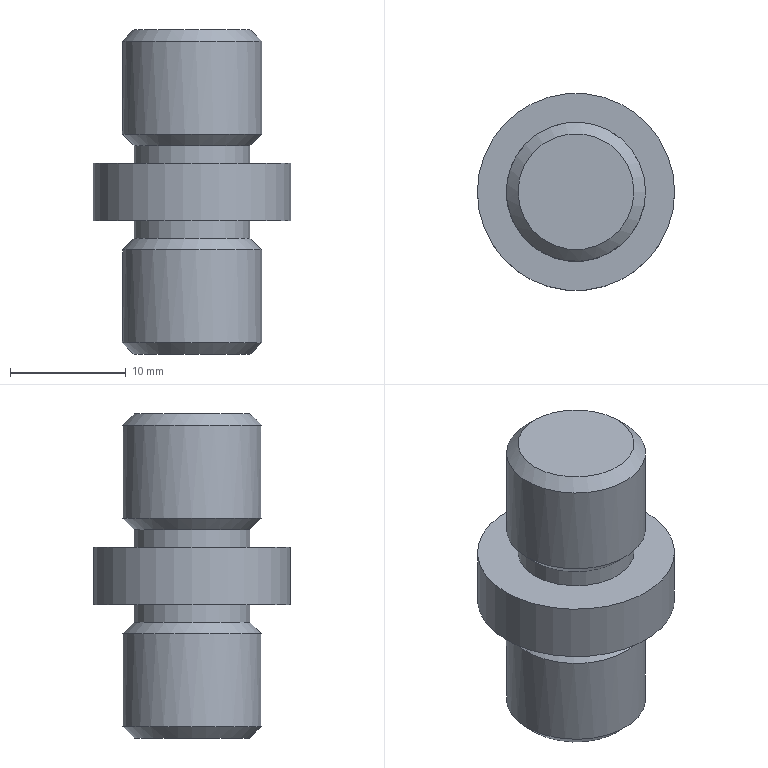Component | NX | A_LOCATING_PIN | 1 solid | 13 faces | box 17 x 17 x 28 mm | volume 3561 mm3 | cylinder 5 | plane 4 | cone 4 | commonest cylinder face diameters 12 x2 10 x2 17 x1
STEP:
#1=CARTESIAN_POINT('',(0.,0.,0.));
#2=DIRECTION('',(0.,0.,1.));
#3=DIRECTION('',(1.,0.,0.));
#4=AXIS2_PLACEMENT_3D('',#1,#2,#3);
#5=CARTESIAN_POINT('',(8.,-18.,40.5));
#6=VERTEX_POINT('',#5);
#7=CARTESIAN_POINT('',(13.,-18.,40.5));
#8=DIRECTION('',(0.,0.,-1.));
#9=DIRECTION('',(-1.,0.,0.));
#10=AXIS2_PLACEMENT_3D('',#7,#8,#9);
#11=CIRCLE('',#10,5.);
#12=CARTESIAN_POINT('',(13.,-18.,40.5));
#13=DIRECTION('',(0.,0.,-1.));
#14=DIRECTION('',(-1.,0.,0.));
#15=AXIS2_PLACEMENT_3D('',#12,#13,#14);
#16=PLANE('',#15);
#17=CARTESIAN_POINT('',(0.,0.));
#18=DIRECTION('',(1.,0.));
#19=AXIS2_PLACEMENT_2D('',#17,#18);
#20=CIRCLE('',#19,5.);
#21=(GEOMETRIC_REPRESENTATION_CONTEXT(2)PARAMETRIC_REPRESENTATION_CONTEXT()REPRESENTATION_CONTEXT('',''));
#22=DEFINITIONAL_REPRESENTATION('',(#20),#21);
#23=PCURVE('',#16,#22);
#24=CARTESIAN_POINT('',(13.,-18.,41.5));
#25=DIRECTION('',(0.,0.,1.));
#26=DIRECTION('',(1.,0.,0.));
#27=AXIS2_PLACEMENT_3D('',#24,#25,#26);
#28=CONICAL_SURFACE('',#27,6.,0.7854);
#29=CARTESIAN_POINT('',(9.425,-1.));
#30=DIRECTION('',(-1.,0.));
#31=VECTOR('',#30,1.);
#32=LINE('',#29,#31);
#33=(GEOMETRIC_REPRESENTATION_CONTEXT(2)PARAMETRIC_REPRESENTATION_CONTEXT()REPRESENTATION_CONTEXT('',''));
#34=DEFINITIONAL_REPRESENTATION('',(#32),#33);
#35=PCURVE('',#28,#34);
#36=SURFACE_CURVE('',#11,(#23,#35),.PCURVE_S1.);
#37=EDGE_CURVE('',#6,#6,#36,.T.);
#38=ORIENTED_EDGE('',*,*,#37,.T.);
#39=EDGE_LOOP('',(#38));
#40=FACE_BOUND('',#39,.T.);
#41=ADVANCED_FACE('',(#40),#16,.T.);
#42=CARTESIAN_POINT('',(7.,-18.,41.5));
#43=VERTEX_POINT('',#42);
#44=CARTESIAN_POINT('',(19.,-18.,41.5));
#45=VERTEX_POINT('',#44);
#46=CARTESIAN_POINT('',(13.,-18.,41.5));
#47=DIRECTION('',(0.,0.,1.));
#48=DIRECTION('',(-1.,0.,0.));
#49=AXIS2_PLACEMENT_3D('',#46,#47,#48);
#50=CIRCLE('',#49,6.);
#51=CARTESIAN_POINT('',(13.,-18.,40.5));
#52=DIRECTION('',(0.,0.,1.));
#53=DIRECTION('',(1.,0.,0.));
#54=AXIS2_PLACEMENT_3D('',#51,#52,#53);
#55=CYLINDRICAL_SURFACE('',#54,6.);
#56=CARTESIAN_POINT('',(3.142,1.));
#57=DIRECTION('',(1.,0.));
#58=VECTOR('',#57,1.);
#59=LINE('',#56,#58);
#60=(GEOMETRIC_REPRESENTATION_CONTEXT(2)PARAMETRIC_REPRESENTATION_CONTEXT()REPRESENTATION_CONTEXT('',''));
#61=DEFINITIONAL_REPRESENTATION('',(#59),#60);
#62=PCURVE('',#55,#61);
#63=CARTESIAN_POINT('',(3.142,0.));
#64=DIRECTION('',(1.,0.));
#65=VECTOR('',#64,1.);
#66=LINE('',#63,#65);
#67=(GEOMETRIC_REPRESENTATION_CONTEXT(2)PARAMETRIC_REPRESENTATION_CONTEXT()REPRESENTATION_CONTEXT('',''));
#68=DEFINITIONAL_REPRESENTATION('',(#66),#67);
#69=PCURVE('',#28,#68);
#70=SURFACE_CURVE('',#50,(#62,#69),.PCURVE_S1.);
#71=EDGE_CURVE('',#43,#45,#70,.T.);
#72=ORIENTED_EDGE('',*,*,#71,.T.);
#73=CARTESIAN_POINT('',(19.,-18.,49.5));
#74=VERTEX_POINT('',#73);
#75=CARTESIAN_POINT('',(19.,-18.,41.5));
#76=CARTESIAN_POINT('',(19.,-18.,49.5));
#77=B_SPLINE_CURVE_WITH_KNOTS('',1,(#75,#76),.UNSPECIFIED.,.F.,.F.,(2,2),(1.,9.),.PIECEWISE_BEZIER_KNOTS.);
#78=CARTESIAN_POINT('',(6.283,0.));
#79=DIRECTION('',(0.,1.));
#80=VECTOR('',#79,1.);
#81=LINE('',#78,#80);
#82=(GEOMETRIC_REPRESENTATION_CONTEXT(2)PARAMETRIC_REPRESENTATION_CONTEXT()REPRESENTATION_CONTEXT('',''));
#83=DEFINITIONAL_REPRESENTATION('',(#81),#82);
#84=PCURVE('',#55,#83);
#85=CARTESIAN_POINT('',(0.,0.));
#86=DIRECTION('',(0.,1.));
#87=VECTOR('',#86,1.);
#88=LINE('',#85,#87);
#89=(GEOMETRIC_REPRESENTATION_CONTEXT(2)PARAMETRIC_REPRESENTATION_CONTEXT()REPRESENTATION_CONTEXT('',''));
#90=DEFINITIONAL_REPRESENTATION('',(#88),#89);
#91=PCURVE('',#55,#90);
#92=SEAM_CURVE('',#77,(#84,#91),.PCURVE_S1.);
#93=EDGE_CURVE('',#45,#74,#92,.T.);
#94=ORIENTED_EDGE('',*,*,#93,.T.);
#95=CARTESIAN_POINT('',(13.,-18.,49.5));
#96=DIRECTION('',(0.,0.,-1.));
#97=DIRECTION('',(1.,0.,0.));
#98=AXIS2_PLACEMENT_3D('',#95,#96,#97);
#99=CIRCLE('',#98,6.);
#100=CARTESIAN_POINT('',(6.283,9.));
#101=DIRECTION('',(-1.,0.));
#102=VECTOR('',#101,1.);
#103=LINE('',#100,#102);
#104=(GEOMETRIC_REPRESENTATION_CONTEXT(2)PARAMETRIC_REPRESENTATION_CONTEXT()REPRESENTATION_CONTEXT('',''));
#105=DEFINITIONAL_REPRESENTATION('',(#103),#104);
#106=PCURVE('',#55,#105);
#107=CARTESIAN_POINT('',(13.,-18.,49.5));
#108=DIRECTION('',(0.,0.,-1.));
#109=DIRECTION('',(-1.,0.,0.));
#110=AXIS2_PLACEMENT_3D('',#107,#108,#109);
#111=CONICAL_SURFACE('',#110,6.,0.7854);
#112=CARTESIAN_POINT('',(3.142,0.));
#113=DIRECTION('',(1.,0.));
#114=VECTOR('',#113,1.);
#115=LINE('',#112,#114);
#116=(GEOMETRIC_REPRESENTATION_CONTEXT(2)PARAMETRIC_REPRESENTATION_CONTEXT()REPRESENTATION_CONTEXT('',''));
#117=DEFINITIONAL_REPRESENTATION('',(#115),#116);
#118=PCURVE('',#111,#117);
#119=SURFACE_CURVE('',#99,(#106,#118),.PCURVE_S1.);
#120=EDGE_CURVE('',#74,#74,#119,.T.);
#121=ORIENTED_EDGE('',*,*,#120,.T.);
#122=ORIENTED_EDGE('',*,*,#93,.F.);
#123=CARTESIAN_POINT('',(13.,-18.,41.5));
#124=DIRECTION('',(0.,0.,1.));
#125=DIRECTION('',(-1.,0.,0.));
#126=AXIS2_PLACEMENT_3D('',#123,#124,#125);
#127=CIRCLE('',#126,6.);
#128=CARTESIAN_POINT('',(-3.142,1.));
#129=DIRECTION('',(1.,0.));
#130=VECTOR('',#129,1.);
#131=LINE('',#128,#130);
#132=(GEOMETRIC_REPRESENTATION_CONTEXT(2)PARAMETRIC_REPRESENTATION_CONTEXT()REPRESENTATION_CONTEXT('',''));
#133=DEFINITIONAL_REPRESENTATION('',(#131),#132);
#134=PCURVE('',#55,#133);
#135=CARTESIAN_POINT('',(3.142,0.));
#136=DIRECTION('',(1.,0.));
#137=VECTOR('',#136,1.);
#138=LINE('',#135,#137);
#139=(GEOMETRIC_REPRESENTATION_CONTEXT(2)PARAMETRIC_REPRESENTATION_CONTEXT()REPRESENTATION_CONTEXT('',''));
#140=DEFINITIONAL_REPRESENTATION('',(#138),#139);
#141=PCURVE('',#28,#140);
#142=SURFACE_CURVE('',#127,(#134,#141),.PCURVE_S1.);
#143=EDGE_CURVE('',#45,#43,#142,.T.);
#144=ORIENTED_EDGE('',*,*,#143,.T.);
#145=EDGE_LOOP('',(#72,#94,#121,#122,#144));
#146=FACE_BOUND('',#145,.T.);
#147=ADVANCED_FACE('',(#146),#55,.T.);
#148=CARTESIAN_POINT('',(18.,-18.,52.));
#149=VERTEX_POINT('',#148);
#150=CARTESIAN_POINT('',(8.,-18.,52.));
#151=VERTEX_POINT('',#150);
#152=CARTESIAN_POINT('',(13.,-18.,52.));
#153=DIRECTION('',(0.,0.,1.));
#154=DIRECTION('',(-1.,0.,0.));
#155=AXIS2_PLACEMENT_3D('',#152,#153,#154);
#156=CIRCLE('',#155,5.);
#157=CARTESIAN_POINT('',(13.,-18.,50.5));
#158=DIRECTION('',(0.,0.,1.));
#159=DIRECTION('',(1.,0.,0.));
#160=AXIS2_PLACEMENT_3D('',#157,#158,#159);
#161=CYLINDRICAL_SURFACE('',#160,5.);
#162=CARTESIAN_POINT('',(-3.142,1.5));
#163=DIRECTION('',(1.,0.));
#164=VECTOR('',#163,1.);
#165=LINE('',#162,#164);
#166=(GEOMETRIC_REPRESENTATION_CONTEXT(2)PARAMETRIC_REPRESENTATION_CONTEXT()REPRESENTATION_CONTEXT('',''));
#167=DEFINITIONAL_REPRESENTATION('',(#165),#166);
#168=PCURVE('',#161,#167);
#169=CARTESIAN_POINT('',(13.,-18.,52.));
#170=DIRECTION('',(0.,0.,-1.));
#171=DIRECTION('',(-1.,0.,0.));
#172=AXIS2_PLACEMENT_3D('',#169,#170,#171);
#173=PLANE('',#172);
#174=CARTESIAN_POINT('',(5.,0.));
#175=CARTESIAN_POINT('',(5.,-8.66));
#176=CARTESIAN_POINT('',(-2.5,-4.33));
#177=CARTESIAN_POINT('',(-10.,-0.));
#178=CARTESIAN_POINT('',(-2.5,4.33));
#179=CARTESIAN_POINT('',(5.,8.66));
#180=CARTESIAN_POINT('',(5.,0.));
#181=(BOUNDED_CURVE()B_SPLINE_CURVE(2,(#174,#175,#176,#177,#178,#179,#180),.UNSPECIFIED.,.T.,.F.)B_SPLINE_CURVE_WITH_KNOTS((1,2,2,2,2,1),(-2.094,0.,2.094,4.189,6.283,8.378),.UNSPECIFIED.)CURVE()GEOMETRIC_REPRESENTATION_ITEM()RATIONAL_B_SPLINE_CURVE((1.,0.5,1.,0.5,1.,0.5,1.))REPRESENTATION_ITEM(''));
#182=(GEOMETRIC_REPRESENTATION_CONTEXT(2)PARAMETRIC_REPRESENTATION_CONTEXT()REPRESENTATION_CONTEXT('',''));
#183=DEFINITIONAL_REPRESENTATION('',(#181),#182);
#184=PCURVE('',#173,#183);
#185=SURFACE_CURVE('',#156,(#168,#184),.PCURVE_S1.);
#186=EDGE_CURVE('',#149,#151,#185,.T.);
#187=ORIENTED_EDGE('',*,*,#186,.F.);
#188=CARTESIAN_POINT('',(18.,-18.,50.5));
#189=VERTEX_POINT('',#188);
#190=CARTESIAN_POINT('',(18.,-18.,50.5));
#191=CARTESIAN_POINT('',(18.,-18.,52.));
#192=B_SPLINE_CURVE_WITH_KNOTS('',1,(#190,#191),.UNSPECIFIED.,.F.,.F.,(2,2),(0.,1.5),.PIECEWISE_BEZIER_KNOTS.);
#193=CARTESIAN_POINT('',(0.,0.));
#194=DIRECTION('',(0.,1.));
#195=VECTOR('',#194,1.);
#196=LINE('',#193,#195);
#197=(GEOMETRIC_REPRESENTATION_CONTEXT(2)PARAMETRIC_REPRESENTATION_CONTEXT()REPRESENTATION_CONTEXT('',''));
#198=DEFINITIONAL_REPRESENTATION('',(#196),#197);
#199=PCURVE('',#161,#198);
#200=CARTESIAN_POINT('',(6.283,0.));
#201=DIRECTION('',(0.,1.));
#202=VECTOR('',#201,1.);
#203=LINE('',#200,#202);
#204=(GEOMETRIC_REPRESENTATION_CONTEXT(2)PARAMETRIC_REPRESENTATION_CONTEXT()REPRESENTATION_CONTEXT('',''));
#205=DEFINITIONAL_REPRESENTATION('',(#203),#204);
#206=PCURVE('',#161,#205);
#207=SEAM_CURVE('',#192,(#199,#206),.PCURVE_S1.);
#208=EDGE_CURVE('',#189,#149,#207,.T.);
#209=ORIENTED_EDGE('',*,*,#208,.F.);
#210=CARTESIAN_POINT('',(13.,-18.,50.5));
#211=DIRECTION('',(0.,0.,1.));
#212=DIRECTION('',(1.,0.,0.));
#213=AXIS2_PLACEMENT_3D('',#210,#211,#212);
#214=CIRCLE('',#213,5.);
#215=CARTESIAN_POINT('',(0.,0.));
#216=DIRECTION('',(1.,0.));
#217=VECTOR('',#216,1.);
#218=LINE('',#215,#217);
#219=(GEOMETRIC_REPRESENTATION_CONTEXT(2)PARAMETRIC_REPRESENTATION_CONTEXT()REPRESENTATION_CONTEXT('',''));
#220=DEFINITIONAL_REPRESENTATION('',(#218),#219);
#221=PCURVE('',#161,#220);
#222=CARTESIAN_POINT('',(9.425,-1.));
#223=DIRECTION('',(-1.,0.));
#224=VECTOR('',#223,1.);
#225=LINE('',#222,#224);
#226=(GEOMETRIC_REPRESENTATION_CONTEXT(2)PARAMETRIC_REPRESENTATION_CONTEXT()REPRESENTATION_CONTEXT('',''));
#227=DEFINITIONAL_REPRESENTATION('',(#225),#226);
#228=PCURVE('',#111,#227);
#229=SURFACE_CURVE('',#214,(#221,#228),.PCURVE_S1.);
#230=EDGE_CURVE('',#189,#189,#229,.T.);
#231=ORIENTED_EDGE('',*,*,#230,.T.);
#232=ORIENTED_EDGE('',*,*,#208,.T.);
#233=CARTESIAN_POINT('',(13.,-18.,52.));
#234=DIRECTION('',(0.,0.,1.));
#235=DIRECTION('',(-1.,0.,0.));
#236=AXIS2_PLACEMENT_3D('',#233,#234,#235);
#237=CIRCLE('',#236,5.);
#238=CARTESIAN_POINT('',(3.142,1.5));
#239=DIRECTION('',(1.,0.));
#240=VECTOR('',#239,1.);
#241=LINE('',#238,#240);
#242=(GEOMETRIC_REPRESENTATION_CONTEXT(2)PARAMETRIC_REPRESENTATION_CONTEXT()REPRESENTATION_CONTEXT('',''));
#243=DEFINITIONAL_REPRESENTATION('',(#241),#242);
#244=PCURVE('',#161,#243);
#245=CARTESIAN_POINT('',(5.,0.));
#246=CARTESIAN_POINT('',(5.,-8.66));
#247=CARTESIAN_POINT('',(-2.5,-4.33));
#248=CARTESIAN_POINT('',(-10.,-0.));
#249=CARTESIAN_POINT('',(-2.5,4.33));
#250=CARTESIAN_POINT('',(5.,8.66));
#251=CARTESIAN_POINT('',(5.,0.));
#252=(BOUNDED_CURVE()B_SPLINE_CURVE(2,(#245,#246,#247,#248,#249,#250,#251),.UNSPECIFIED.,.T.,.F.)B_SPLINE_CURVE_WITH_KNOTS((1,2,2,2,2,1),(-2.094,0.,2.094,4.189,6.283,8.378),.UNSPECIFIED.)CURVE()GEOMETRIC_REPRESENTATION_ITEM()RATIONAL_B_SPLINE_CURVE((1.,0.5,1.,0.5,1.,0.5,1.))REPRESENTATION_ITEM(''));
#253=(GEOMETRIC_REPRESENTATION_CONTEXT(2)PARAMETRIC_REPRESENTATION_CONTEXT()REPRESENTATION_CONTEXT('',''));
#254=DEFINITIONAL_REPRESENTATION('',(#252),#253);
#255=PCURVE('',#173,#254);
#256=SURFACE_CURVE('',#237,(#244,#255),.PCURVE_S1.);
#257=EDGE_CURVE('',#151,#149,#256,.T.);
#258=ORIENTED_EDGE('',*,*,#257,.F.);
#259=EDGE_LOOP('',(#187,#209,#231,#232,#258));
#260=FACE_BOUND('',#259,.T.);
#261=ADVANCED_FACE('',(#260),#161,.T.);
#262=CARTESIAN_POINT('',(18.,-18.,57.));
#263=VERTEX_POINT('',#262);
#264=CARTESIAN_POINT('',(13.,-18.,57.));
#265=DIRECTION('',(0.,0.,1.));
#266=DIRECTION('',(1.,0.,0.));
#267=AXIS2_PLACEMENT_3D('',#264,#265,#266);
#268=CIRCLE('',#267,5.);
#269=CARTESIAN_POINT('',(13.,-18.,57.));
#270=DIRECTION('',(0.,0.,1.));
#271=DIRECTION('',(1.,0.,0.));
#272=AXIS2_PLACEMENT_3D('',#269,#270,#271);
#273=PLANE('',#272);
#274=CARTESIAN_POINT('',(0.,0.));
#275=DIRECTION('',(1.,0.));
#276=AXIS2_PLACEMENT_2D('',#274,#275);
#277=CIRCLE('',#276,5.);
#278=(GEOMETRIC_REPRESENTATION_CONTEXT(2)PARAMETRIC_REPRESENTATION_CONTEXT()REPRESENTATION_CONTEXT('',''));
#279=DEFINITIONAL_REPRESENTATION('',(#277),#278);
#280=PCURVE('',#273,#279);
#281=CARTESIAN_POINT('',(13.,-18.,57.));
#282=DIRECTION('',(0.,0.,1.));
#283=DIRECTION('',(1.,0.,0.));
#284=AXIS2_PLACEMENT_3D('',#281,#282,#283);
#285=CYLINDRICAL_SURFACE('',#284,5.);
#286=CARTESIAN_POINT('',(0.,0.));
#287=DIRECTION('',(1.,0.));
#288=VECTOR('',#287,1.);
#289=LINE('',#286,#288);
#290=(GEOMETRIC_REPRESENTATION_CONTEXT(2)PARAMETRIC_REPRESENTATION_CONTEXT()REPRESENTATION_CONTEXT('',''));
#291=DEFINITIONAL_REPRESENTATION('',(#289),#290);
#292=PCURVE('',#285,#291);
#293=SURFACE_CURVE('',#268,(#280,#292),.PCURVE_S1.);
#294=EDGE_CURVE('',#263,#263,#293,.T.);
#295=ORIENTED_EDGE('',*,*,#294,.F.);
#296=EDGE_LOOP('',(#295));
#297=FACE_BOUND('',#296,.T.);
#298=CARTESIAN_POINT('',(21.5,-18.,57.));
#299=VERTEX_POINT('',#298);
#300=CARTESIAN_POINT('',(13.,-18.,57.));
#301=DIRECTION('',(0.,0.,-1.));
#302=DIRECTION('',(1.,0.,0.));
#303=AXIS2_PLACEMENT_3D('',#300,#301,#302);
#304=CIRCLE('',#303,8.5);
#305=CARTESIAN_POINT('',(8.5,0.));
#306=CARTESIAN_POINT('',(8.5,-14.722));
#307=CARTESIAN_POINT('',(-4.25,-7.361));
#308=CARTESIAN_POINT('',(-17.,-0.));
#309=CARTESIAN_POINT('',(-4.25,7.361));
#310=CARTESIAN_POINT('',(8.5,14.722));
#311=CARTESIAN_POINT('',(8.5,0.));
#312=(BOUNDED_CURVE()B_SPLINE_CURVE(2,(#305,#306,#307,#308,#309,#310,#311),.UNSPECIFIED.,.T.,.F.)B_SPLINE_CURVE_WITH_KNOTS((1,2,2,2,2,1),(-2.094,0.,2.094,4.189,6.283,8.378),.UNSPECIFIED.)CURVE()GEOMETRIC_REPRESENTATION_ITEM()RATIONAL_B_SPLINE_CURVE((1.,0.5,1.,0.5,1.,0.5,1.))REPRESENTATION_ITEM(''));
#313=(GEOMETRIC_REPRESENTATION_CONTEXT(2)PARAMETRIC_REPRESENTATION_CONTEXT()REPRESENTATION_CONTEXT('',''));
#314=DEFINITIONAL_REPRESENTATION('',(#312),#313);
#315=PCURVE('',#273,#314);
#316=CARTESIAN_POINT('',(13.,-18.,52.));
#317=DIRECTION('',(0.,0.,1.));
#318=DIRECTION('',(1.,0.,0.));
#319=AXIS2_PLACEMENT_3D('',#316,#317,#318);
#320=CYLINDRICAL_SURFACE('',#319,8.5);
#321=CARTESIAN_POINT('',(6.283,5.));
#322=DIRECTION('',(-1.,0.));
#323=VECTOR('',#322,1.);
#324=LINE('',#321,#323);
#325=(GEOMETRIC_REPRESENTATION_CONTEXT(2)PARAMETRIC_REPRESENTATION_CONTEXT()REPRESENTATION_CONTEXT('',''));
#326=DEFINITIONAL_REPRESENTATION('',(#324),#325);
#327=PCURVE('',#320,#326);
#328=SURFACE_CURVE('',#304,(#315,#327),.PCURVE_S1.);
#329=EDGE_CURVE('',#299,#299,#328,.T.);
#330=ORIENTED_EDGE('',*,*,#329,.F.);
#331=EDGE_LOOP('',(#330));
#332=FACE_BOUND('',#331,.T.);
#333=ADVANCED_FACE('',(#297,#332),#273,.T.);
#334=ORIENTED_EDGE('',*,*,#257,.T.);
#335=ORIENTED_EDGE('',*,*,#186,.T.);
#336=EDGE_LOOP('',(#334,#335));
#337=FACE_BOUND('',#336,.T.);
#338=CARTESIAN_POINT('',(21.5,-18.,52.));
#339=VERTEX_POINT('',#338);
#340=CARTESIAN_POINT('',(13.,-18.,52.));
#341=DIRECTION('',(0.,0.,1.));
#342=DIRECTION('',(1.,0.,0.));
#343=AXIS2_PLACEMENT_3D('',#340,#341,#342);
#344=CIRCLE('',#343,8.5);
#345=CARTESIAN_POINT('',(-8.5,0.));
#346=CARTESIAN_POINT('',(-8.5,14.722));
#347=CARTESIAN_POINT('',(4.25,7.361));
#348=CARTESIAN_POINT('',(17.,0.));
#349=CARTESIAN_POINT('',(4.25,-7.361));
#350=CARTESIAN_POINT('',(-8.5,-14.722));
#351=CARTESIAN_POINT('',(-8.5,0.));
#352=(BOUNDED_CURVE()B_SPLINE_CURVE(2,(#345,#346,#347,#348,#349,#350,#351),.UNSPECIFIED.,.T.,.F.)B_SPLINE_CURVE_WITH_KNOTS((1,2,2,2,2,1),(-2.094,0.,2.094,4.189,6.283,8.378),.UNSPECIFIED.)CURVE()GEOMETRIC_REPRESENTATION_ITEM()RATIONAL_B_SPLINE_CURVE((1.,0.5,1.,0.5,1.,0.5,1.))REPRESENTATION_ITEM(''));
#353=(GEOMETRIC_REPRESENTATION_CONTEXT(2)PARAMETRIC_REPRESENTATION_CONTEXT()REPRESENTATION_CONTEXT('',''));
#354=DEFINITIONAL_REPRESENTATION('',(#352),#353);
#355=PCURVE('',#173,#354);
#356=CARTESIAN_POINT('',(0.,0.));
#357=DIRECTION('',(1.,0.));
#358=VECTOR('',#357,1.);
#359=LINE('',#356,#358);
#360=(GEOMETRIC_REPRESENTATION_CONTEXT(2)PARAMETRIC_REPRESENTATION_CONTEXT()REPRESENTATION_CONTEXT('',''));
#361=DEFINITIONAL_REPRESENTATION('',(#359),#360);
#362=PCURVE('',#320,#361);
#363=SURFACE_CURVE('',#344,(#355,#362),.PCURVE_S1.);
#364=EDGE_CURVE('',#339,#339,#363,.T.);
#365=ORIENTED_EDGE('',*,*,#364,.F.);
#366=EDGE_LOOP('',(#365));
#367=FACE_BOUND('',#366,.T.);
#368=ADVANCED_FACE('',(#337,#367),#173,.T.);
#369=ORIENTED_EDGE('',*,*,#329,.T.);
#370=CARTESIAN_POINT('',(21.5,-18.,52.));
#371=CARTESIAN_POINT('',(21.5,-18.,57.));
#372=B_SPLINE_CURVE_WITH_KNOTS('',1,(#370,#371),.UNSPECIFIED.,.F.,.F.,(2,2),(0.,5.),.PIECEWISE_BEZIER_KNOTS.);
#373=CARTESIAN_POINT('',(0.,0.));
#374=DIRECTION('',(0.,1.));
#375=VECTOR('',#374,1.);
#376=LINE('',#373,#375);
#377=(GEOMETRIC_REPRESENTATION_CONTEXT(2)PARAMETRIC_REPRESENTATION_CONTEXT()REPRESENTATION_CONTEXT('',''));
#378=DEFINITIONAL_REPRESENTATION('',(#376),#377);
#379=PCURVE('',#320,#378);
#380=CARTESIAN_POINT('',(6.283,0.));
#381=DIRECTION('',(0.,1.));
#382=VECTOR('',#381,1.);
#383=LINE('',#380,#382);
#384=(GEOMETRIC_REPRESENTATION_CONTEXT(2)PARAMETRIC_REPRESENTATION_CONTEXT()REPRESENTATION_CONTEXT('',''));
#385=DEFINITIONAL_REPRESENTATION('',(#383),#384);
#386=PCURVE('',#320,#385);
#387=SEAM_CURVE('',#372,(#379,#386),.PCURVE_S1.);
#388=EDGE_CURVE('',#339,#299,#387,.T.);
#389=ORIENTED_EDGE('',*,*,#388,.F.);
#390=ORIENTED_EDGE('',*,*,#364,.T.);
#391=ORIENTED_EDGE('',*,*,#388,.T.);
#392=EDGE_LOOP('',(#369,#389,#390,#391));
#393=FACE_BOUND('',#392,.T.);
#394=ADVANCED_FACE('',(#393),#320,.T.);
#395=CARTESIAN_POINT('',(18.,-18.,58.5));
#396=VERTEX_POINT('',#395);
#397=CARTESIAN_POINT('',(8.,-18.,58.5));
#398=VERTEX_POINT('',#397);
#399=CARTESIAN_POINT('',(13.,-18.,58.5));
#400=DIRECTION('',(0.,0.,1.));
#401=DIRECTION('',(-1.,0.,0.));
#402=AXIS2_PLACEMENT_3D('',#399,#400,#401);
#403=CIRCLE('',#402,5.);
#404=CARTESIAN_POINT('',(-3.142,1.5));
#405=DIRECTION('',(1.,0.));
#406=VECTOR('',#405,1.);
#407=LINE('',#404,#406);
#408=(GEOMETRIC_REPRESENTATION_CONTEXT(2)PARAMETRIC_REPRESENTATION_CONTEXT()REPRESENTATION_CONTEXT('',''));
#409=DEFINITIONAL_REPRESENTATION('',(#407),#408);
#410=PCURVE('',#285,#409);
#411=CARTESIAN_POINT('',(13.,-18.,59.5));
#412=DIRECTION('',(0.,0.,1.));
#413=DIRECTION('',(1.,0.,0.));
#414=AXIS2_PLACEMENT_3D('',#411,#412,#413);
#415=CONICAL_SURFACE('',#414,6.,0.7854);
#416=CARTESIAN_POINT('',(-3.142,-1.));
#417=DIRECTION('',(1.,0.));
#418=VECTOR('',#417,1.);
#419=LINE('',#416,#418);
#420=(GEOMETRIC_REPRESENTATION_CONTEXT(2)PARAMETRIC_REPRESENTATION_CONTEXT()REPRESENTATION_CONTEXT('',''));
#421=DEFINITIONAL_REPRESENTATION('',(#419),#420);
#422=PCURVE('',#415,#421);
#423=SURFACE_CURVE('',#403,(#410,#422),.PCURVE_S1.);
#424=EDGE_CURVE('',#396,#398,#423,.T.);
#425=ORIENTED_EDGE('',*,*,#424,.F.);
#426=CARTESIAN_POINT('',(18.,-18.,57.));
#427=CARTESIAN_POINT('',(18.,-18.,58.5));
#428=B_SPLINE_CURVE_WITH_KNOTS('',1,(#426,#427),.UNSPECIFIED.,.F.,.F.,(2,2),(0.,1.5),.PIECEWISE_BEZIER_KNOTS.);
#429=CARTESIAN_POINT('',(0.,0.));
#430=DIRECTION('',(0.,1.));
#431=VECTOR('',#430,1.);
#432=LINE('',#429,#431);
#433=(GEOMETRIC_REPRESENTATION_CONTEXT(2)PARAMETRIC_REPRESENTATION_CONTEXT()REPRESENTATION_CONTEXT('',''));
#434=DEFINITIONAL_REPRESENTATION('',(#432),#433);
#435=PCURVE('',#285,#434);
#436=CARTESIAN_POINT('',(6.283,0.));
#437=DIRECTION('',(0.,1.));
#438=VECTOR('',#437,1.);
#439=LINE('',#436,#438);
#440=(GEOMETRIC_REPRESENTATION_CONTEXT(2)PARAMETRIC_REPRESENTATION_CONTEXT()REPRESENTATION_CONTEXT('',''));
#441=DEFINITIONAL_REPRESENTATION('',(#439),#440);
#442=PCURVE('',#285,#441);
#443=SEAM_CURVE('',#428,(#435,#442),.PCURVE_S1.);
#444=EDGE_CURVE('',#263,#396,#443,.T.);
#445=ORIENTED_EDGE('',*,*,#444,.F.);
#446=ORIENTED_EDGE('',*,*,#294,.T.);
#447=ORIENTED_EDGE('',*,*,#444,.T.);
#448=CARTESIAN_POINT('',(13.,-18.,58.5));
#449=DIRECTION('',(0.,0.,1.));
#450=DIRECTION('',(-1.,0.,0.));
#451=AXIS2_PLACEMENT_3D('',#448,#449,#450);
#452=CIRCLE('',#451,5.);
#453=CARTESIAN_POINT('',(3.142,1.5));
#454=DIRECTION('',(1.,0.));
#455=VECTOR('',#454,1.);
#456=LINE('',#453,#455);
#457=(GEOMETRIC_REPRESENTATION_CONTEXT(2)PARAMETRIC_REPRESENTATION_CONTEXT()REPRESENTATION_CONTEXT('',''));
#458=DEFINITIONAL_REPRESENTATION('',(#456),#457);
#459=PCURVE('',#285,#458);
#460=CARTESIAN_POINT('',(3.142,-1.));
#461=DIRECTION('',(1.,0.));
#462=VECTOR('',#461,1.);
#463=LINE('',#460,#462);
#464=(GEOMETRIC_REPRESENTATION_CONTEXT(2)PARAMETRIC_REPRESENTATION_CONTEXT()REPRESENTATION_CONTEXT('',''));
#465=DEFINITIONAL_REPRESENTATION('',(#463),#464);
#466=PCURVE('',#415,#465);
#467=SURFACE_CURVE('',#452,(#459,#466),.PCURVE_S1.);
#468=EDGE_CURVE('',#398,#396,#467,.T.);
#469=ORIENTED_EDGE('',*,*,#468,.F.);
#470=EDGE_LOOP('',(#425,#445,#446,#447,#469));
#471=FACE_BOUND('',#470,.T.);
#472=ADVANCED_FACE('',(#471),#285,.T.);
#473=CARTESIAN_POINT('',(18.,-18.,68.5));
#474=VERTEX_POINT('',#473);
#475=CARTESIAN_POINT('',(13.,-18.,68.5));
#476=DIRECTION('',(0.,0.,1.));
#477=DIRECTION('',(1.,0.,0.));
#478=AXIS2_PLACEMENT_3D('',#475,#476,#477);
#479=CIRCLE('',#478,5.);
#480=CARTESIAN_POINT('',(13.,-18.,68.5));
#481=DIRECTION('',(0.,0.,1.));
#482=DIRECTION('',(1.,0.,0.));
#483=AXIS2_PLACEMENT_3D('',#480,#481,#482);
#484=PLANE('',#483);
#485=CARTESIAN_POINT('',(0.,0.));
#486=DIRECTION('',(1.,0.));
#487=AXIS2_PLACEMENT_2D('',#485,#486);
#488=CIRCLE('',#487,5.);
#489=(GEOMETRIC_REPRESENTATION_CONTEXT(2)PARAMETRIC_REPRESENTATION_CONTEXT()REPRESENTATION_CONTEXT('',''));
#490=DEFINITIONAL_REPRESENTATION('',(#488),#489);
#491=PCURVE('',#484,#490);
#492=CARTESIAN_POINT('',(13.,-18.,67.5));
#493=DIRECTION('',(0.,0.,-1.));
#494=DIRECTION('',(-1.,0.,0.));
#495=AXIS2_PLACEMENT_3D('',#492,#493,#494);
#496=CONICAL_SURFACE('',#495,6.,0.7854);
#497=CARTESIAN_POINT('',(9.425,-1.));
#498=DIRECTION('',(-1.,0.));
#499=VECTOR('',#498,1.);
#500=LINE('',#497,#499);
#501=(GEOMETRIC_REPRESENTATION_CONTEXT(2)PARAMETRIC_REPRESENTATION_CONTEXT()REPRESENTATION_CONTEXT('',''));
#502=DEFINITIONAL_REPRESENTATION('',(#500),#501);
#503=PCURVE('',#496,#502);
#504=SURFACE_CURVE('',#479,(#491,#503),.PCURVE_S1.);
#505=EDGE_CURVE('',#474,#474,#504,.T.);
#506=ORIENTED_EDGE('',*,*,#505,.T.);
#507=EDGE_LOOP('',(#506));
#508=FACE_BOUND('',#507,.T.);
#509=ADVANCED_FACE('',(#508),#484,.T.);
#510=CARTESIAN_POINT('',(7.,-18.,59.5));
#511=VERTEX_POINT('',#510);
#512=CARTESIAN_POINT('',(19.,-18.,59.5));
#513=VERTEX_POINT('',#512);
#514=CARTESIAN_POINT('',(13.,-18.,59.5));
#515=DIRECTION('',(0.,0.,1.));
#516=DIRECTION('',(-1.,0.,0.));
#517=AXIS2_PLACEMENT_3D('',#514,#515,#516);
#518=CIRCLE('',#517,6.);
#519=CARTESIAN_POINT('',(13.,-18.,58.5));
#520=DIRECTION('',(0.,0.,1.));
#521=DIRECTION('',(1.,0.,0.));
#522=AXIS2_PLACEMENT_3D('',#519,#520,#521);
#523=CYLINDRICAL_SURFACE('',#522,6.);
#524=CARTESIAN_POINT('',(3.142,1.));
#525=DIRECTION('',(1.,0.));
#526=VECTOR('',#525,1.);
#527=LINE('',#524,#526);
#528=(GEOMETRIC_REPRESENTATION_CONTEXT(2)PARAMETRIC_REPRESENTATION_CONTEXT()REPRESENTATION_CONTEXT('',''));
#529=DEFINITIONAL_REPRESENTATION('',(#527),#528);
#530=PCURVE('',#523,#529);
#531=CARTESIAN_POINT('',(3.142,0.));
#532=DIRECTION('',(1.,0.));
#533=VECTOR('',#532,1.);
#534=LINE('',#531,#533);
#535=(GEOMETRIC_REPRESENTATION_CONTEXT(2)PARAMETRIC_REPRESENTATION_CONTEXT()REPRESENTATION_CONTEXT('',''));
#536=DEFINITIONAL_REPRESENTATION('',(#534),#535);
#537=PCURVE('',#415,#536);
#538=SURFACE_CURVE('',#518,(#530,#537),.PCURVE_S1.);
#539=EDGE_CURVE('',#511,#513,#538,.T.);
#540=ORIENTED_EDGE('',*,*,#539,.T.);
#541=CARTESIAN_POINT('',(19.,-18.,67.5));
#542=VERTEX_POINT('',#541);
#543=CARTESIAN_POINT('',(19.,-18.,59.5));
#544=CARTESIAN_POINT('',(19.,-18.,67.5));
#545=B_SPLINE_CURVE_WITH_KNOTS('',1,(#543,#544),.UNSPECIFIED.,.F.,.F.,(2,2),(1.,9.),.PIECEWISE_BEZIER_KNOTS.);
#546=CARTESIAN_POINT('',(6.283,0.));
#547=DIRECTION('',(0.,1.));
#548=VECTOR('',#547,1.);
#549=LINE('',#546,#548);
#550=(GEOMETRIC_REPRESENTATION_CONTEXT(2)PARAMETRIC_REPRESENTATION_CONTEXT()REPRESENTATION_CONTEXT('',''));
#551=DEFINITIONAL_REPRESENTATION('',(#549),#550);
#552=PCURVE('',#523,#551);
#553=CARTESIAN_POINT('',(0.,0.));
#554=DIRECTION('',(0.,1.));
#555=VECTOR('',#554,1.);
#556=LINE('',#553,#555);
#557=(GEOMETRIC_REPRESENTATION_CONTEXT(2)PARAMETRIC_REPRESENTATION_CONTEXT()REPRESENTATION_CONTEXT('',''));
#558=DEFINITIONAL_REPRESENTATION('',(#556),#557);
#559=PCURVE('',#523,#558);
#560=SEAM_CURVE('',#545,(#552,#559),.PCURVE_S1.);
#561=EDGE_CURVE('',#513,#542,#560,.T.);
#562=ORIENTED_EDGE('',*,*,#561,.T.);
#563=CARTESIAN_POINT('',(13.,-18.,67.5));
#564=DIRECTION('',(0.,0.,-1.));
#565=DIRECTION('',(1.,0.,0.));
#566=AXIS2_PLACEMENT_3D('',#563,#564,#565);
#567=CIRCLE('',#566,6.);
#568=CARTESIAN_POINT('',(6.283,9.));
#569=DIRECTION('',(-1.,0.));
#570=VECTOR('',#569,1.);
#571=LINE('',#568,#570);
#572=(GEOMETRIC_REPRESENTATION_CONTEXT(2)PARAMETRIC_REPRESENTATION_CONTEXT()REPRESENTATION_CONTEXT('',''));
#573=DEFINITIONAL_REPRESENTATION('',(#571),#572);
#574=PCURVE('',#523,#573);
#575=CARTESIAN_POINT('',(3.142,0.));
#576=DIRECTION('',(1.,0.));
#577=VECTOR('',#576,1.);
#578=LINE('',#575,#577);
#579=(GEOMETRIC_REPRESENTATION_CONTEXT(2)PARAMETRIC_REPRESENTATION_CONTEXT()REPRESENTATION_CONTEXT('',''));
#580=DEFINITIONAL_REPRESENTATION('',(#578),#579);
#581=PCURVE('',#496,#580);
#582=SURFACE_CURVE('',#567,(#574,#581),.PCURVE_S1.);
#583=EDGE_CURVE('',#542,#542,#582,.T.);
#584=ORIENTED_EDGE('',*,*,#583,.T.);
#585=ORIENTED_EDGE('',*,*,#561,.F.);
#586=CARTESIAN_POINT('',(13.,-18.,59.5));
#587=DIRECTION('',(0.,0.,1.));
#588=DIRECTION('',(-1.,0.,0.));
#589=AXIS2_PLACEMENT_3D('',#586,#587,#588);
#590=CIRCLE('',#589,6.);
#591=CARTESIAN_POINT('',(-3.142,1.));
#592=DIRECTION('',(1.,0.));
#593=VECTOR('',#592,1.);
#594=LINE('',#591,#593);
#595=(GEOMETRIC_REPRESENTATION_CONTEXT(2)PARAMETRIC_REPRESENTATION_CONTEXT()REPRESENTATION_CONTEXT('',''));
#596=DEFINITIONAL_REPRESENTATION('',(#594),#595);
#597=PCURVE('',#523,#596);
#598=CARTESIAN_POINT('',(-3.142,0.));
#599=DIRECTION('',(1.,0.));
#600=VECTOR('',#599,1.);
#601=LINE('',#598,#600);
#602=(GEOMETRIC_REPRESENTATION_CONTEXT(2)PARAMETRIC_REPRESENTATION_CONTEXT()REPRESENTATION_CONTEXT('',''));
#603=DEFINITIONAL_REPRESENTATION('',(#601),#602);
#604=PCURVE('',#415,#603);
#605=SURFACE_CURVE('',#590,(#597,#604),.PCURVE_S1.);
#606=EDGE_CURVE('',#513,#511,#605,.T.);
#607=ORIENTED_EDGE('',*,*,#606,.T.);
#608=EDGE_LOOP('',(#540,#562,#584,#585,#607));
#609=FACE_BOUND('',#608,.T.);
#610=ADVANCED_FACE('',(#609),#523,.T.);
#611=ORIENTED_EDGE('',*,*,#37,.F.);
#612=CARTESIAN_POINT('',(8.,-18.,40.5));
#613=CARTESIAN_POINT('',(7.,-18.,41.5));
#614=B_SPLINE_CURVE_WITH_KNOTS('',1,(#612,#613),.UNSPECIFIED.,.F.,.F.,(2,2),(-1.414,0.),.PIECEWISE_BEZIER_KNOTS.);
#615=CARTESIAN_POINT('',(9.425,0.));
#616=DIRECTION('',(0.,1.));
#617=VECTOR('',#616,1.);
#618=LINE('',#615,#617);
#619=(GEOMETRIC_REPRESENTATION_CONTEXT(2)PARAMETRIC_REPRESENTATION_CONTEXT()REPRESENTATION_CONTEXT('',''));
#620=DEFINITIONAL_REPRESENTATION('',(#618),#619);
#621=PCURVE('',#28,#620);
#622=CARTESIAN_POINT('',(3.142,0.));
#623=DIRECTION('',(0.,1.));
#624=VECTOR('',#623,1.);
#625=LINE('',#622,#624);
#626=(GEOMETRIC_REPRESENTATION_CONTEXT(2)PARAMETRIC_REPRESENTATION_CONTEXT()REPRESENTATION_CONTEXT('',''));
#627=DEFINITIONAL_REPRESENTATION('',(#625),#626);
#628=PCURVE('',#28,#627);
#629=SEAM_CURVE('',#614,(#621,#628),.PCURVE_S1.);
#630=EDGE_CURVE('',#6,#43,#629,.T.);
#631=ORIENTED_EDGE('',*,*,#630,.T.);
#632=ORIENTED_EDGE('',*,*,#143,.F.);
#633=ORIENTED_EDGE('',*,*,#71,.F.);
#634=ORIENTED_EDGE('',*,*,#630,.F.);
#635=EDGE_LOOP('',(#611,#631,#632,#633,#634));
#636=FACE_BOUND('',#635,.T.);
#637=ADVANCED_FACE('',(#636),#28,.T.);
#638=ORIENTED_EDGE('',*,*,#230,.F.);
#639=CARTESIAN_POINT('',(18.,-18.,50.5));
#640=CARTESIAN_POINT('',(19.,-18.,49.5));
#641=B_SPLINE_CURVE_WITH_KNOTS('',1,(#639,#640),.UNSPECIFIED.,.F.,.F.,(2,2),(-1.414,0.),.PIECEWISE_BEZIER_KNOTS.);
#642=CARTESIAN_POINT('',(9.425,0.));
#643=DIRECTION('',(0.,1.));
#644=VECTOR('',#643,1.);
#645=LINE('',#642,#644);
#646=(GEOMETRIC_REPRESENTATION_CONTEXT(2)PARAMETRIC_REPRESENTATION_CONTEXT()REPRESENTATION_CONTEXT('',''));
#647=DEFINITIONAL_REPRESENTATION('',(#645),#646);
#648=PCURVE('',#111,#647);
#649=CARTESIAN_POINT('',(3.142,0.));
#650=DIRECTION('',(0.,1.));
#651=VECTOR('',#650,1.);
#652=LINE('',#649,#651);
#653=(GEOMETRIC_REPRESENTATION_CONTEXT(2)PARAMETRIC_REPRESENTATION_CONTEXT()REPRESENTATION_CONTEXT('',''));
#654=DEFINITIONAL_REPRESENTATION('',(#652),#653);
#655=PCURVE('',#111,#654);
#656=SEAM_CURVE('',#641,(#648,#655),.PCURVE_S1.);
#657=EDGE_CURVE('',#189,#74,#656,.T.);
#658=ORIENTED_EDGE('',*,*,#657,.T.);
#659=ORIENTED_EDGE('',*,*,#120,.F.);
#660=ORIENTED_EDGE('',*,*,#657,.F.);
#661=EDGE_LOOP('',(#638,#658,#659,#660));
#662=FACE_BOUND('',#661,.T.);
#663=ADVANCED_FACE('',(#662),#111,.T.);
#664=ORIENTED_EDGE('',*,*,#468,.T.);
#665=CARTESIAN_POINT('',(18.,-18.,58.5));
#666=CARTESIAN_POINT('',(19.,-18.,59.5));
#667=B_SPLINE_CURVE_WITH_KNOTS('',1,(#665,#666),.UNSPECIFIED.,.F.,.F.,(2,2),(-1.414,0.),.PIECEWISE_BEZIER_KNOTS.);
#668=CARTESIAN_POINT('',(6.283,0.));
#669=DIRECTION('',(0.,1.));
#670=VECTOR('',#669,1.);
#671=LINE('',#668,#670);
#672=(GEOMETRIC_REPRESENTATION_CONTEXT(2)PARAMETRIC_REPRESENTATION_CONTEXT()REPRESENTATION_CONTEXT('',''));
#673=DEFINITIONAL_REPRESENTATION('',(#671),#672);
#674=PCURVE('',#415,#673);
#675=CARTESIAN_POINT('',(0.,0.));
#676=DIRECTION('',(0.,1.));
#677=VECTOR('',#676,1.);
#678=LINE('',#675,#677);
#679=(GEOMETRIC_REPRESENTATION_CONTEXT(2)PARAMETRIC_REPRESENTATION_CONTEXT()REPRESENTATION_CONTEXT('',''));
#680=DEFINITIONAL_REPRESENTATION('',(#678),#679);
#681=PCURVE('',#415,#680);
#682=SEAM_CURVE('',#667,(#674,#681),.PCURVE_S1.);
#683=EDGE_CURVE('',#396,#513,#682,.T.);
#684=ORIENTED_EDGE('',*,*,#683,.T.);
#685=ORIENTED_EDGE('',*,*,#539,.F.);
#686=ORIENTED_EDGE('',*,*,#606,.F.);
#687=ORIENTED_EDGE('',*,*,#683,.F.);
#688=ORIENTED_EDGE('',*,*,#424,.T.);
#689=EDGE_LOOP('',(#664,#684,#685,#686,#687,#688));
#690=FACE_BOUND('',#689,.T.);
#691=ADVANCED_FACE('',(#690),#415,.T.);
#692=ORIENTED_EDGE('',*,*,#505,.F.);
#693=CARTESIAN_POINT('',(18.,-18.,68.5));
#694=CARTESIAN_POINT('',(19.,-18.,67.5));
#695=B_SPLINE_CURVE_WITH_KNOTS('',1,(#693,#694),.UNSPECIFIED.,.F.,.F.,(2,2),(-1.414,0.),.PIECEWISE_BEZIER_KNOTS.);
#696=CARTESIAN_POINT('',(9.425,0.));
#697=DIRECTION('',(0.,1.));
#698=VECTOR('',#697,1.);
#699=LINE('',#696,#698);
#700=(GEOMETRIC_REPRESENTATION_CONTEXT(2)PARAMETRIC_REPRESENTATION_CONTEXT()REPRESENTATION_CONTEXT('',''));
#701=DEFINITIONAL_REPRESENTATION('',(#699),#700);
#702=PCURVE('',#496,#701);
#703=CARTESIAN_POINT('',(3.142,0.));
#704=DIRECTION('',(0.,1.));
#705=VECTOR('',#704,1.);
#706=LINE('',#703,#705);
#707=(GEOMETRIC_REPRESENTATION_CONTEXT(2)PARAMETRIC_REPRESENTATION_CONTEXT()REPRESENTATION_CONTEXT('',''));
#708=DEFINITIONAL_REPRESENTATION('',(#706),#707);
#709=PCURVE('',#496,#708);
#710=SEAM_CURVE('',#695,(#702,#709),.PCURVE_S1.);
#711=EDGE_CURVE('',#474,#542,#710,.T.);
#712=ORIENTED_EDGE('',*,*,#711,.T.);
#713=ORIENTED_EDGE('',*,*,#583,.F.);
#714=ORIENTED_EDGE('',*,*,#711,.F.);
#715=EDGE_LOOP('',(#692,#712,#713,#714));
#716=FACE_BOUND('',#715,.T.);
#717=ADVANCED_FACE('',(#716),#496,.T.);
#718=CLOSED_SHELL('',(#41,#147,#261,#333,#368,#394,#472,#509,#610,#637,#663,#691,#717));
#719=MANIFOLD_SOLID_BREP('',#718);
#720=(LENGTH_UNIT()NAMED_UNIT(*)SI_UNIT(.MILLI.,.METRE.));
#721=UNCERTAINTY_MEASURE_WITH_UNIT(LENGTH_MEASURE(0.000005),#720,'','');
#722=(NAMED_UNIT(*)PLANE_ANGLE_UNIT()SI_UNIT($,.RADIAN.));
#723=(NAMED_UNIT(*)SI_UNIT($,.STERADIAN.)SOLID_ANGLE_UNIT());
#724=(GEOMETRIC_REPRESENTATION_CONTEXT(3)GLOBAL_UNCERTAINTY_ASSIGNED_CONTEXT((#721))GLOBAL_UNIT_ASSIGNED_CONTEXT((#720,#722,#723))REPRESENTATION_CONTEXT('',''));
#725=ADVANCED_BREP_SHAPE_REPRESENTATION('',(#4,#719),#724);